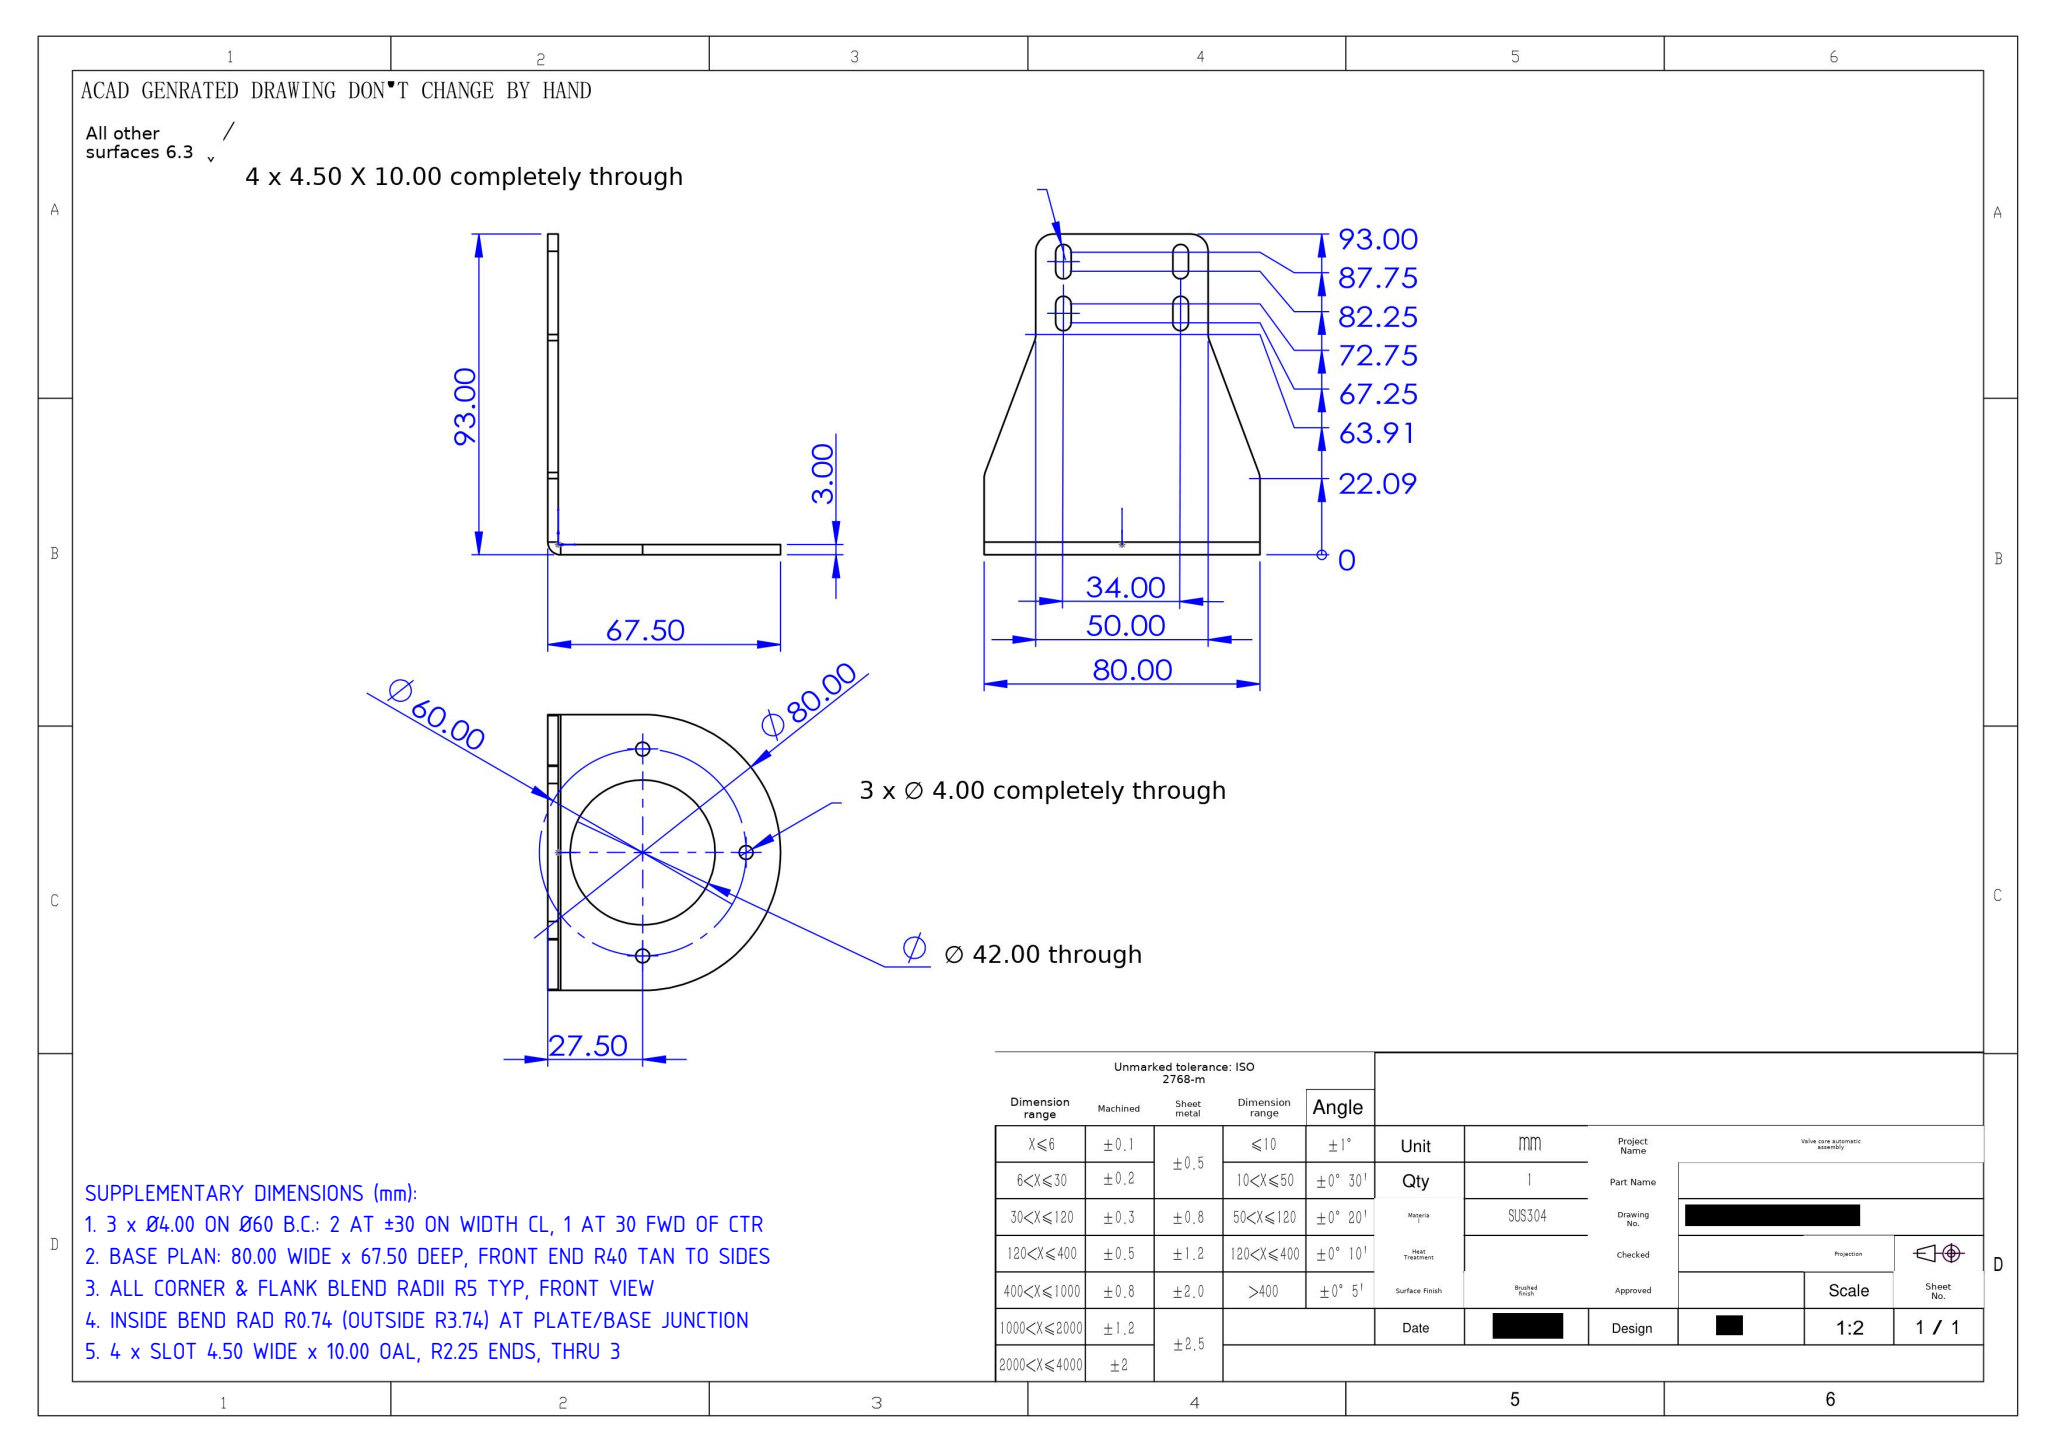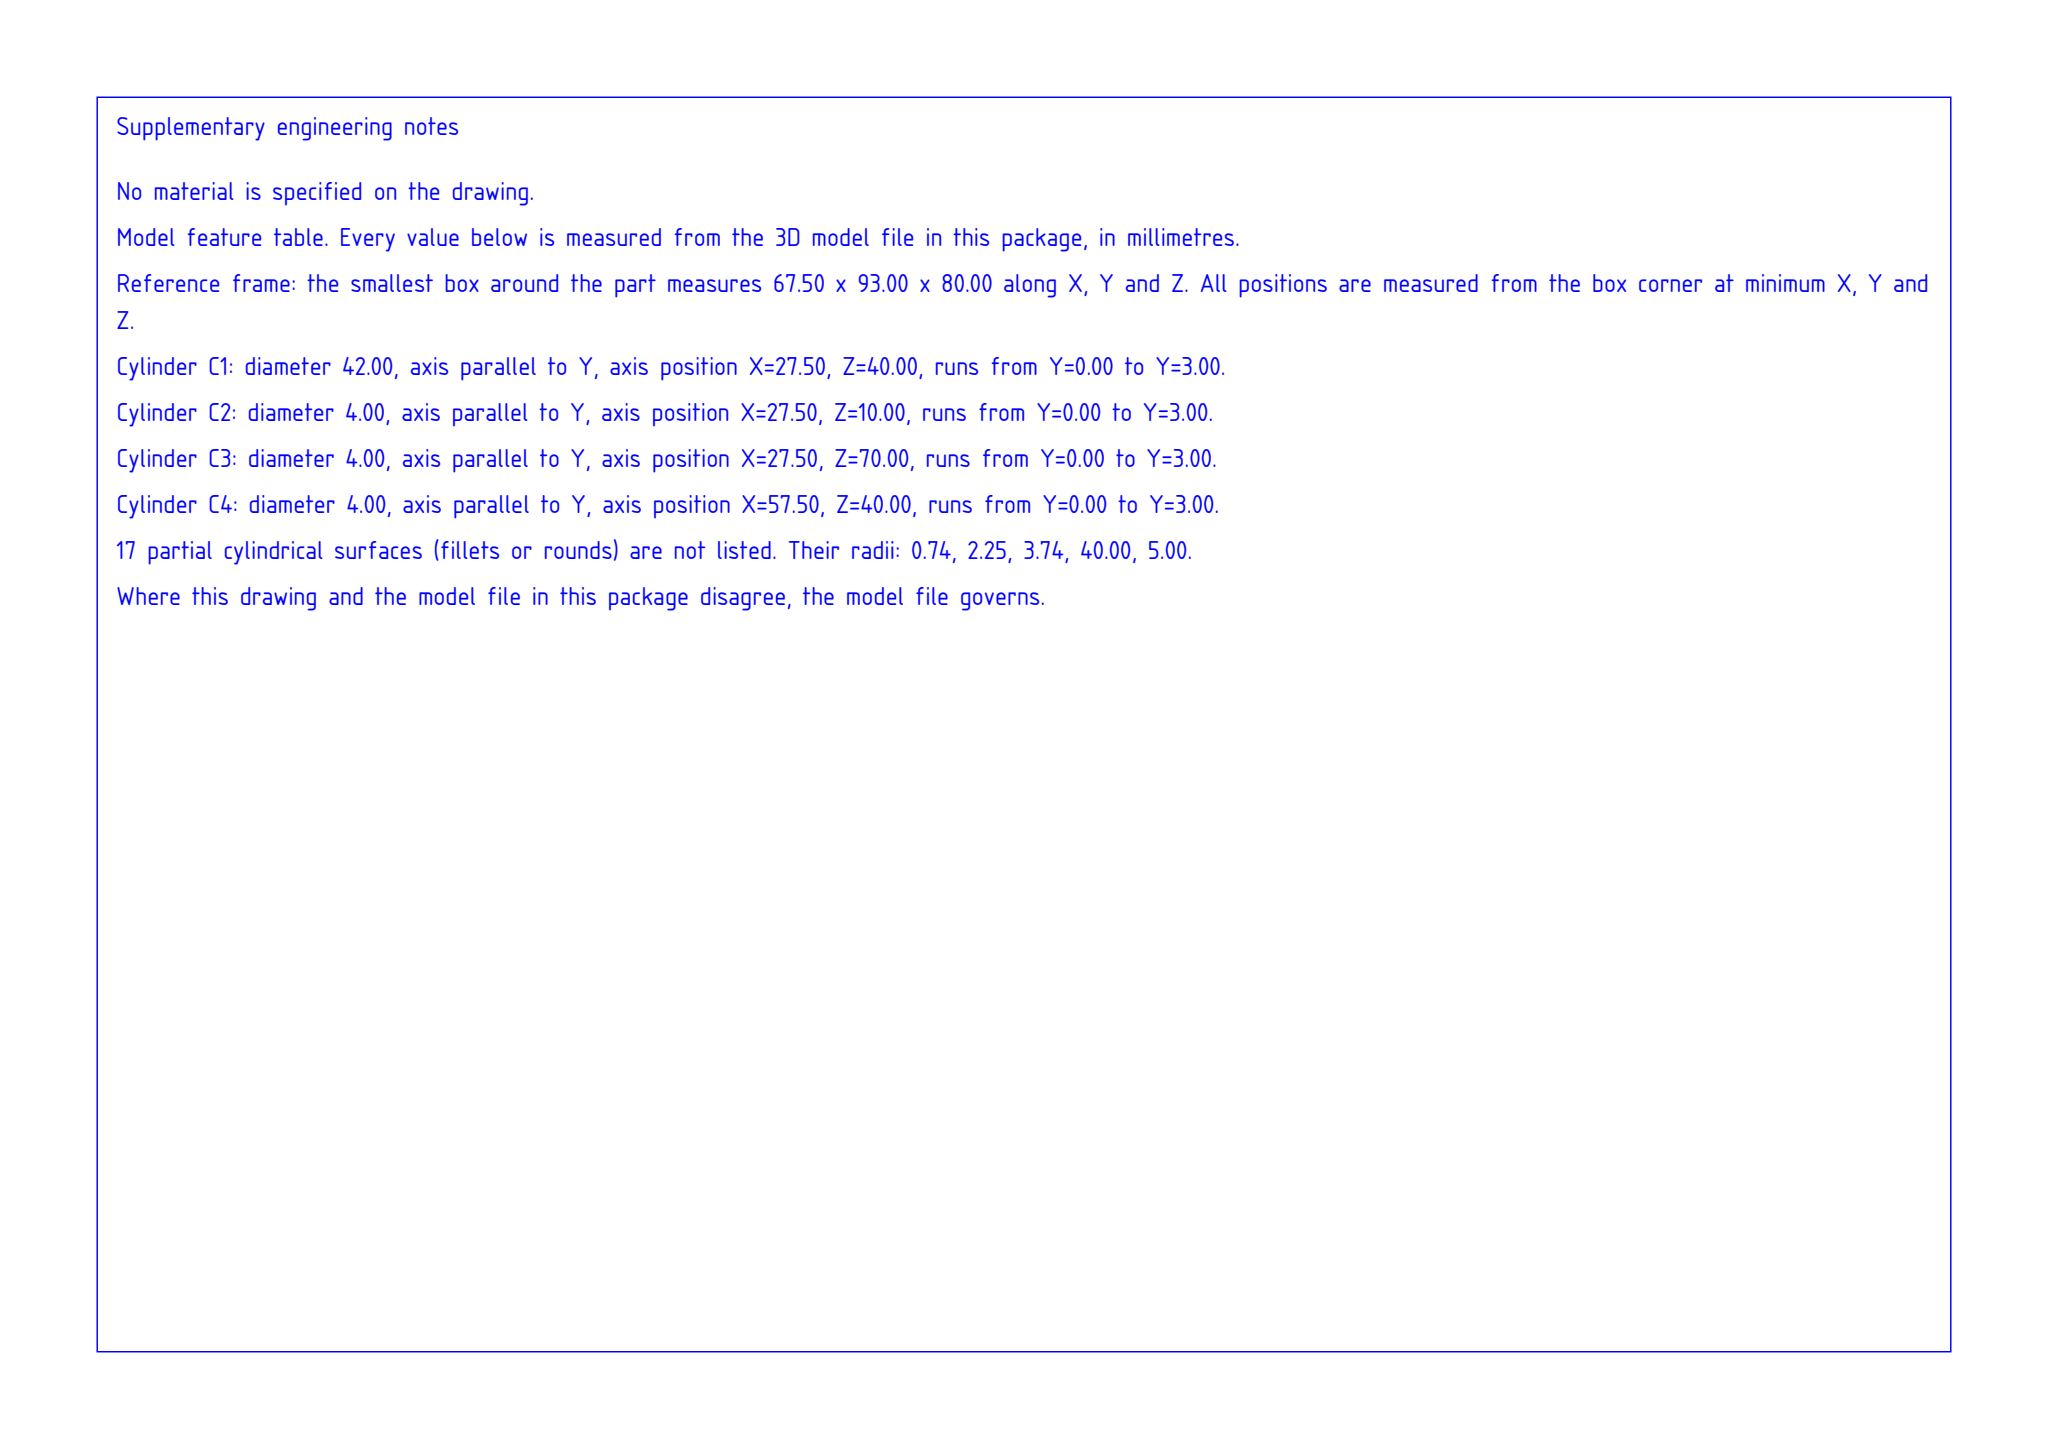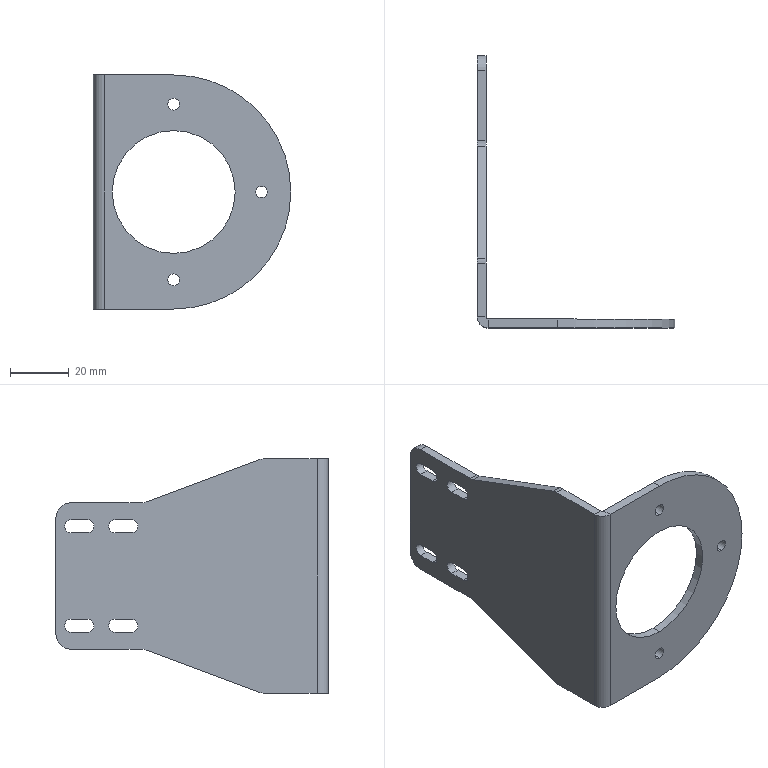Part | SolidWorks | mm | 1 solid | 53 faces | box 67.5 x 93 x 80 mm | volume 26220 mm3 | cylinder 30 | plane 23 | commonest cylinder face diameters 4.5 x12 4 x6 10 x6 42 x2 80 x2 1.473 x1 7.473 x1